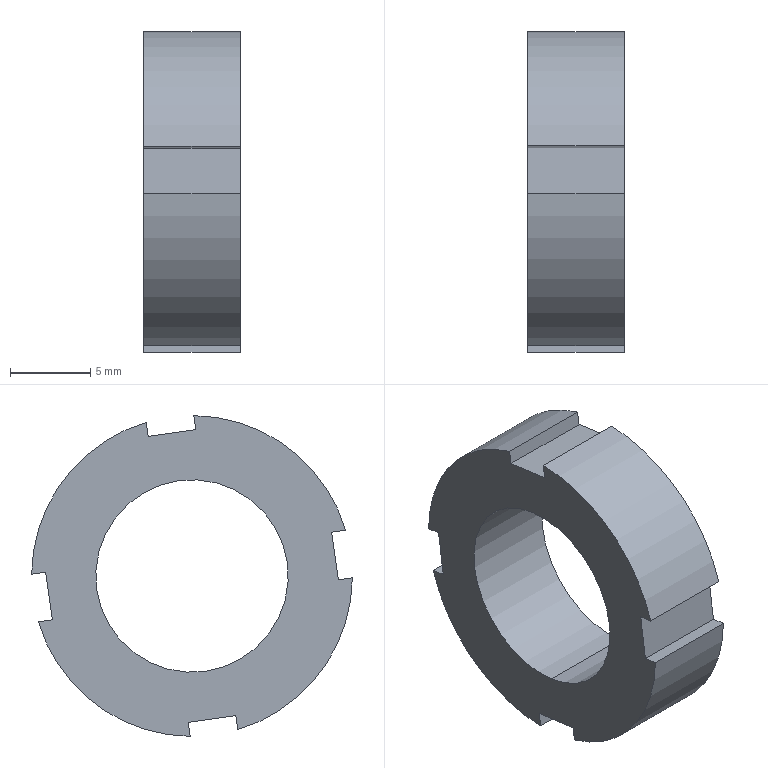Component | SolidWorks | ElectricalBoxAssembly2-1_RoundNut-1 | 1 solid | 20 faces | box 6 x 20 x 20 mm | volume 1137 mm3 | plane 14 | cylinder 6 | commonest cylinder face diameters 20 x4 12 x2
STEP:
#1=COLOUR_RGB('',0.7922,0.8196,0.9333);
#2=FILL_AREA_STYLE_COLOUR('',#1);
#3=FILL_AREA_STYLE('',(#2));
#4=SURFACE_STYLE_FILL_AREA(#3);
#5=SURFACE_SIDE_STYLE('',(#4));
#6=SURFACE_STYLE_USAGE(.BOTH.,#5);
#7=PRESENTATION_STYLE_ASSIGNMENT((#6));
#8=CARTESIAN_POINT('',(29.585,8.484,66.234));
#9=VERTEX_POINT('',#8);
#10=CARTESIAN_POINT('',(29.585,8.419,65.766));
#11=VERTEX_POINT('',#10);
#12=CARTESIAN_POINT('',(29.585,8.451,66.));
#13=DIRECTION('',(-1.,-0.,-0.));
#14=DIRECTION('',(0.,-0.1386,-0.9903));
#15=AXIS2_PLACEMENT_3D('',#12,#13,#14);
#16=CIRCLE('',#15,0.2362);
#17=EDGE_CURVE('',#9,#11,#16,.T.);
#18=ORIENTED_EDGE('',*,*,#17,.T.);
#19=CARTESIAN_POINT('',(29.822,8.419,65.766));
#20=VERTEX_POINT('',#19);
#21=CARTESIAN_POINT('',(29.585,8.419,65.766));
#22=DIRECTION('',(1.,0.,0.));
#23=VECTOR('',#22,39.37);
#24=LINE('',#21,#23);
#25=EDGE_CURVE('',#11,#20,#24,.T.);
#26=ORIENTED_EDGE('',*,*,#25,.T.);
#27=CARTESIAN_POINT('',(29.822,8.484,66.234));
#28=VERTEX_POINT('',#27);
#29=CARTESIAN_POINT('',(29.822,8.451,66.));
#30=DIRECTION('',(-1.,-0.,-0.));
#31=DIRECTION('',(0.,-0.1386,-0.9903));
#32=AXIS2_PLACEMENT_3D('',#29,#30,#31);
#33=CIRCLE('',#32,0.2362);
#34=EDGE_CURVE('',#28,#20,#33,.T.);
#35=ORIENTED_EDGE('',*,*,#34,.F.);
#36=CARTESIAN_POINT('',(29.585,8.484,66.234));
#37=DIRECTION('',(1.,0.,0.));
#38=VECTOR('',#37,39.37);
#39=LINE('',#36,#38);
#40=EDGE_CURVE('',#9,#28,#39,.T.);
#41=ORIENTED_EDGE('',*,*,#40,.F.);
#42=EDGE_LOOP('',(#18,#26,#35,#41));
#43=FACE_OUTER_BOUND('',#42,.T.);
#44=CARTESIAN_POINT('',(29.585,8.451,66.));
#45=DIRECTION('',(1.,0.,0.));
#46=DIRECTION('',(0.,0.1386,0.9903));
#47=AXIS2_PLACEMENT_3D('',#44,#45,#46);
#48=CYLINDRICAL_SURFACE('',#47,0.2362);
#49=ADVANCED_FACE('',(#43),#48,.F.);
#50=CARTESIAN_POINT('',(29.822,8.564,66.377));
#51=VERTEX_POINT('',#50);
#52=CARTESIAN_POINT('',(29.822,8.845,66.004));
#53=VERTEX_POINT('',#52);
#54=CARTESIAN_POINT('',(29.822,8.451,66.));
#55=DIRECTION('',(-1.,-0.,-0.));
#56=DIRECTION('',(0.,-0.1386,-0.9903));
#57=AXIS2_PLACEMENT_3D('',#54,#55,#56);
#58=CIRCLE('',#57,0.3937);
#59=EDGE_CURVE('',#51,#53,#58,.T.);
#60=ORIENTED_EDGE('',*,*,#59,.T.);
#61=CARTESIAN_POINT('',(29.585,8.845,66.004));
#62=VERTEX_POINT('',#61);
#63=CARTESIAN_POINT('',(29.585,8.845,66.004));
#64=DIRECTION('',(-1.,-0.,-0.));
#65=VECTOR('',#64,39.37);
#66=LINE('',#63,#65);
#67=EDGE_CURVE('',#53,#62,#66,.T.);
#68=ORIENTED_EDGE('',*,*,#67,.T.);
#69=CARTESIAN_POINT('',(29.585,8.564,66.377));
#70=VERTEX_POINT('',#69);
#71=CARTESIAN_POINT('',(29.585,8.451,66.));
#72=DIRECTION('',(-1.,-0.,-0.));
#73=DIRECTION('',(0.,-0.1386,-0.9903));
#74=AXIS2_PLACEMENT_3D('',#71,#72,#73);
#75=CIRCLE('',#74,0.3937);
#76=EDGE_CURVE('',#70,#62,#75,.T.);
#77=ORIENTED_EDGE('',*,*,#76,.F.);
#78=CARTESIAN_POINT('',(29.585,8.564,66.377));
#79=DIRECTION('',(1.,0.,0.));
#80=VECTOR('',#79,39.37);
#81=LINE('',#78,#80);
#82=EDGE_CURVE('',#70,#51,#81,.T.);
#83=ORIENTED_EDGE('',*,*,#82,.T.);
#84=EDGE_LOOP('',(#60,#68,#77,#83));
#85=FACE_OUTER_BOUND('',#84,.T.);
#86=CARTESIAN_POINT('',(29.585,8.451,66.));
#87=DIRECTION('',(1.,0.,0.));
#88=DIRECTION('',(0.,0.1386,0.9903));
#89=AXIS2_PLACEMENT_3D('',#86,#87,#88);
#90=CYLINDRICAL_SURFACE('',#89,0.3937);
#91=ADVANCED_FACE('',(#85),#90,.T.);
#92=CARTESIAN_POINT('',(29.822,8.074,66.112));
#93=VERTEX_POINT('',#92);
#94=CARTESIAN_POINT('',(29.822,8.447,66.394));
#95=VERTEX_POINT('',#94);
#96=CARTESIAN_POINT('',(29.822,8.451,66.));
#97=DIRECTION('',(-1.,-0.,-0.));
#98=DIRECTION('',(0.,-0.1386,-0.9903));
#99=AXIS2_PLACEMENT_3D('',#96,#97,#98);
#100=CIRCLE('',#99,0.3937);
#101=EDGE_CURVE('',#93,#95,#100,.T.);
#102=ORIENTED_EDGE('',*,*,#101,.T.);
#103=CARTESIAN_POINT('',(29.585,8.447,66.394));
#104=VERTEX_POINT('',#103);
#105=CARTESIAN_POINT('',(29.585,8.447,66.394));
#106=DIRECTION('',(-1.,-0.,-0.));
#107=VECTOR('',#106,39.37);
#108=LINE('',#105,#107);
#109=EDGE_CURVE('',#95,#104,#108,.T.);
#110=ORIENTED_EDGE('',*,*,#109,.T.);
#111=CARTESIAN_POINT('',(29.585,8.074,66.112));
#112=VERTEX_POINT('',#111);
#113=CARTESIAN_POINT('',(29.585,8.451,66.));
#114=DIRECTION('',(-1.,-0.,-0.));
#115=DIRECTION('',(0.,-0.1386,-0.9903));
#116=AXIS2_PLACEMENT_3D('',#113,#114,#115);
#117=CIRCLE('',#116,0.3937);
#118=EDGE_CURVE('',#112,#104,#117,.T.);
#119=ORIENTED_EDGE('',*,*,#118,.F.);
#120=CARTESIAN_POINT('',(29.585,8.074,66.112));
#121=DIRECTION('',(1.,0.,0.));
#122=VECTOR('',#121,39.37);
#123=LINE('',#120,#122);
#124=EDGE_CURVE('',#112,#93,#123,.T.);
#125=ORIENTED_EDGE('',*,*,#124,.T.);
#126=EDGE_LOOP('',(#102,#110,#119,#125));
#127=FACE_OUTER_BOUND('',#126,.T.);
#128=CARTESIAN_POINT('',(29.585,8.451,66.));
#129=DIRECTION('',(1.,0.,0.));
#130=DIRECTION('',(0.,0.1386,0.9903));
#131=AXIS2_PLACEMENT_3D('',#128,#129,#130);
#132=CYLINDRICAL_SURFACE('',#131,0.3937);
#133=ADVANCED_FACE('',(#127),#132,.T.);
#134=CARTESIAN_POINT('',(29.585,8.829,65.888));
#135=VERTEX_POINT('',#134);
#136=CARTESIAN_POINT('',(29.585,8.456,65.606));
#137=VERTEX_POINT('',#136);
#138=CARTESIAN_POINT('',(29.585,8.451,66.));
#139=DIRECTION('',(-1.,-0.,-0.));
#140=DIRECTION('',(0.,-0.1386,-0.9903));
#141=AXIS2_PLACEMENT_3D('',#138,#139,#140);
#142=CIRCLE('',#141,0.3937);
#143=EDGE_CURVE('',#135,#137,#142,.T.);
#144=ORIENTED_EDGE('',*,*,#143,.F.);
#145=CARTESIAN_POINT('',(29.822,8.829,65.888));
#146=VERTEX_POINT('',#145);
#147=CARTESIAN_POINT('',(29.585,8.829,65.888));
#148=DIRECTION('',(1.,0.,0.));
#149=VECTOR('',#148,39.37);
#150=LINE('',#147,#149);
#151=EDGE_CURVE('',#135,#146,#150,.T.);
#152=ORIENTED_EDGE('',*,*,#151,.T.);
#153=CARTESIAN_POINT('',(29.822,8.456,65.606));
#154=VERTEX_POINT('',#153);
#155=CARTESIAN_POINT('',(29.822,8.451,66.));
#156=DIRECTION('',(-1.,-0.,-0.));
#157=DIRECTION('',(0.,-0.1386,-0.9903));
#158=AXIS2_PLACEMENT_3D('',#155,#156,#157);
#159=CIRCLE('',#158,0.3937);
#160=EDGE_CURVE('',#146,#154,#159,.T.);
#161=ORIENTED_EDGE('',*,*,#160,.T.);
#162=CARTESIAN_POINT('',(29.585,8.456,65.606));
#163=DIRECTION('',(-1.,-0.,-0.));
#164=VECTOR('',#163,39.37);
#165=LINE('',#162,#164);
#166=EDGE_CURVE('',#154,#137,#165,.T.);
#167=ORIENTED_EDGE('',*,*,#166,.T.);
#168=EDGE_LOOP('',(#144,#152,#161,#167));
#169=FACE_OUTER_BOUND('',#168,.T.);
#170=CARTESIAN_POINT('',(29.585,8.451,66.));
#171=DIRECTION('',(1.,0.,0.));
#172=DIRECTION('',(0.,0.1386,0.9903));
#173=AXIS2_PLACEMENT_3D('',#170,#171,#172);
#174=CYLINDRICAL_SURFACE('',#173,0.3937);
#175=ADVANCED_FACE('',(#169),#174,.T.);
#176=CARTESIAN_POINT('',(29.585,8.811,66.009));
#177=VERTEX_POINT('',#176);
#178=CARTESIAN_POINT('',(29.585,8.888,65.998));
#179=DIRECTION('',(0.,0.9903,-0.1386));
#180=VECTOR('',#179,39.37);
#181=LINE('',#178,#180);
#182=EDGE_CURVE('',#177,#62,#181,.T.);
#183=ORIENTED_EDGE('',*,*,#182,.F.);
#184=CARTESIAN_POINT('',(29.585,8.794,65.892));
#185=VERTEX_POINT('',#184);
#186=CARTESIAN_POINT('',(29.585,8.794,65.892));
#187=DIRECTION('',(-0.,0.1386,0.9903));
#188=VECTOR('',#187,39.37);
#189=LINE('',#186,#188);
#190=EDGE_CURVE('',#185,#177,#189,.T.);
#191=ORIENTED_EDGE('',*,*,#190,.F.);
#192=CARTESIAN_POINT('',(29.585,8.872,65.881));
#193=DIRECTION('',(-0.,-0.9903,0.1386));
#194=VECTOR('',#193,39.37);
#195=LINE('',#192,#194);
#196=EDGE_CURVE('',#135,#185,#195,.T.);
#197=ORIENTED_EDGE('',*,*,#196,.F.);
#198=ORIENTED_EDGE('',*,*,#143,.T.);
#199=CARTESIAN_POINT('',(29.585,8.461,65.641));
#200=VERTEX_POINT('',#199);
#201=CARTESIAN_POINT('',(29.585,8.45,65.563));
#202=DIRECTION('',(0.,-0.1386,-0.9903));
#203=VECTOR('',#202,39.37);
#204=LINE('',#201,#203);
#205=EDGE_CURVE('',#200,#137,#204,.T.);
#206=ORIENTED_EDGE('',*,*,#205,.F.);
#207=CARTESIAN_POINT('',(29.585,8.344,65.657));
#208=VERTEX_POINT('',#207);
#209=CARTESIAN_POINT('',(29.585,8.344,65.657));
#210=DIRECTION('',(0.,0.9903,-0.1386));
#211=VECTOR('',#210,39.37);
#212=LINE('',#209,#211);
#213=EDGE_CURVE('',#208,#200,#212,.T.);
#214=ORIENTED_EDGE('',*,*,#213,.F.);
#215=CARTESIAN_POINT('',(29.585,8.339,65.623));
#216=VERTEX_POINT('',#215);
#217=CARTESIAN_POINT('',(29.585,8.333,65.579));
#218=DIRECTION('',(-0.,0.1386,0.9903));
#219=VECTOR('',#218,39.37);
#220=LINE('',#217,#219);
#221=EDGE_CURVE('',#216,#208,#220,.T.);
#222=ORIENTED_EDGE('',*,*,#221,.F.);
#223=CARTESIAN_POINT('',(29.585,8.058,65.995));
#224=VERTEX_POINT('',#223);
#225=CARTESIAN_POINT('',(29.585,8.451,66.));
#226=DIRECTION('',(-1.,-0.,-0.));
#227=DIRECTION('',(0.,-0.1386,-0.9903));
#228=AXIS2_PLACEMENT_3D('',#225,#226,#227);
#229=CIRCLE('',#228,0.3937);
#230=EDGE_CURVE('',#216,#224,#229,.T.);
#231=ORIENTED_EDGE('',*,*,#230,.T.);
#232=CARTESIAN_POINT('',(29.585,8.092,65.991));
#233=VERTEX_POINT('',#232);
#234=CARTESIAN_POINT('',(29.585,8.014,66.001));
#235=DIRECTION('',(-0.,-0.9903,0.1386));
#236=VECTOR('',#235,39.37);
#237=LINE('',#234,#236);
#238=EDGE_CURVE('',#233,#224,#237,.T.);
#239=ORIENTED_EDGE('',*,*,#238,.F.);
#240=CARTESIAN_POINT('',(29.585,8.109,66.108));
#241=VERTEX_POINT('',#240);
#242=CARTESIAN_POINT('',(29.585,8.109,66.108));
#243=DIRECTION('',(0.,-0.1386,-0.9903));
#244=VECTOR('',#243,39.37);
#245=LINE('',#242,#244);
#246=EDGE_CURVE('',#241,#233,#245,.T.);
#247=ORIENTED_EDGE('',*,*,#246,.F.);
#248=CARTESIAN_POINT('',(29.585,8.031,66.118));
#249=DIRECTION('',(0.,0.9903,-0.1386));
#250=VECTOR('',#249,39.37);
#251=LINE('',#248,#250);
#252=EDGE_CURVE('',#112,#241,#251,.T.);
#253=ORIENTED_EDGE('',*,*,#252,.F.);
#254=ORIENTED_EDGE('',*,*,#118,.T.);
#255=CARTESIAN_POINT('',(29.585,8.442,66.359));
#256=VERTEX_POINT('',#255);
#257=CARTESIAN_POINT('',(29.585,8.453,66.437));
#258=DIRECTION('',(-0.,0.1386,0.9903));
#259=VECTOR('',#258,39.37);
#260=LINE('',#257,#259);
#261=EDGE_CURVE('',#256,#104,#260,.T.);
#262=ORIENTED_EDGE('',*,*,#261,.F.);
#263=CARTESIAN_POINT('',(29.585,8.559,66.343));
#264=VERTEX_POINT('',#263);
#265=CARTESIAN_POINT('',(29.585,8.559,66.343));
#266=DIRECTION('',(-0.,-0.9903,0.1386));
#267=VECTOR('',#266,39.37);
#268=LINE('',#265,#267);
#269=EDGE_CURVE('',#264,#256,#268,.T.);
#270=ORIENTED_EDGE('',*,*,#269,.F.);
#271=CARTESIAN_POINT('',(29.585,8.57,66.421));
#272=DIRECTION('',(0.,-0.1386,-0.9903));
#273=VECTOR('',#272,39.37);
#274=LINE('',#271,#273);
#275=EDGE_CURVE('',#70,#264,#274,.T.);
#276=ORIENTED_EDGE('',*,*,#275,.F.);
#277=ORIENTED_EDGE('',*,*,#76,.T.);
#278=EDGE_LOOP('',(#183,#191,#197,#198,#206,#214,#222,#231,#239,#247,#253,#254,#262,#270,#276,#277));
#279=FACE_OUTER_BOUND('',#278,.T.);
#280=ORIENTED_EDGE('',*,*,#17,.F.);
#281=CARTESIAN_POINT('',(29.585,8.451,66.));
#282=DIRECTION('',(-1.,-0.,-0.));
#283=DIRECTION('',(0.,-0.1386,-0.9903));
#284=AXIS2_PLACEMENT_3D('',#281,#282,#283);
#285=CIRCLE('',#284,0.2362);
#286=EDGE_CURVE('',#11,#9,#285,.T.);
#287=ORIENTED_EDGE('',*,*,#286,.F.);
#288=EDGE_LOOP('',(#280,#287));
#289=FACE_BOUND('',#288,.T.);
#290=CARTESIAN_POINT('',(29.585,8.451,66.));
#291=DIRECTION('',(-1.,-0.,-0.));
#292=DIRECTION('',(0.,-0.1386,-0.9903));
#293=AXIS2_PLACEMENT_3D('',#290,#291,#292);
#294=PLANE('',#293);
#295=ADVANCED_FACE('',(#279,#289),#294,.T.);
#296=CARTESIAN_POINT('',(29.822,8.794,65.892));
#297=VERTEX_POINT('',#296);
#298=CARTESIAN_POINT('',(29.822,8.811,66.009));
#299=VERTEX_POINT('',#298);
#300=CARTESIAN_POINT('',(29.822,8.794,65.892));
#301=DIRECTION('',(-0.,0.1386,0.9903));
#302=VECTOR('',#301,39.37);
#303=LINE('',#300,#302);
#304=EDGE_CURVE('',#297,#299,#303,.T.);
#305=ORIENTED_EDGE('',*,*,#304,.T.);
#306=CARTESIAN_POINT('',(29.822,8.888,65.998));
#307=DIRECTION('',(0.,0.9903,-0.1386));
#308=VECTOR('',#307,39.37);
#309=LINE('',#306,#308);
#310=EDGE_CURVE('',#299,#53,#309,.T.);
#311=ORIENTED_EDGE('',*,*,#310,.T.);
#312=ORIENTED_EDGE('',*,*,#59,.F.);
#313=CARTESIAN_POINT('',(29.822,8.559,66.343));
#314=VERTEX_POINT('',#313);
#315=CARTESIAN_POINT('',(29.822,8.51,65.992));
#316=DIRECTION('',(0.,-0.1386,-0.9903));
#317=VECTOR('',#316,39.37);
#318=LINE('',#315,#317);
#319=EDGE_CURVE('',#51,#314,#318,.T.);
#320=ORIENTED_EDGE('',*,*,#319,.T.);
#321=CARTESIAN_POINT('',(29.822,8.442,66.359));
#322=VERTEX_POINT('',#321);
#323=CARTESIAN_POINT('',(29.822,8.559,66.343));
#324=DIRECTION('',(-0.,-0.9903,0.1386));
#325=VECTOR('',#324,39.37);
#326=LINE('',#323,#325);
#327=EDGE_CURVE('',#314,#322,#326,.T.);
#328=ORIENTED_EDGE('',*,*,#327,.T.);
#329=CARTESIAN_POINT('',(29.822,8.453,66.437));
#330=DIRECTION('',(-0.,0.1386,0.9903));
#331=VECTOR('',#330,39.37);
#332=LINE('',#329,#331);
#333=EDGE_CURVE('',#322,#95,#332,.T.);
#334=ORIENTED_EDGE('',*,*,#333,.T.);
#335=ORIENTED_EDGE('',*,*,#101,.F.);
#336=CARTESIAN_POINT('',(29.822,8.109,66.108));
#337=VERTEX_POINT('',#336);
#338=CARTESIAN_POINT('',(29.822,8.031,66.118));
#339=DIRECTION('',(0.,0.9903,-0.1386));
#340=VECTOR('',#339,39.37);
#341=LINE('',#338,#340);
#342=EDGE_CURVE('',#93,#337,#341,.T.);
#343=ORIENTED_EDGE('',*,*,#342,.T.);
#344=CARTESIAN_POINT('',(29.822,8.092,65.991));
#345=VERTEX_POINT('',#344);
#346=CARTESIAN_POINT('',(29.822,8.109,66.108));
#347=DIRECTION('',(0.,-0.1386,-0.9903));
#348=VECTOR('',#347,39.37);
#349=LINE('',#346,#348);
#350=EDGE_CURVE('',#337,#345,#349,.T.);
#351=ORIENTED_EDGE('',*,*,#350,.T.);
#352=CARTESIAN_POINT('',(29.822,8.058,65.995));
#353=VERTEX_POINT('',#352);
#354=CARTESIAN_POINT('',(29.822,8.014,66.001));
#355=DIRECTION('',(-0.,-0.9903,0.1386));
#356=VECTOR('',#355,39.37);
#357=LINE('',#354,#356);
#358=EDGE_CURVE('',#345,#353,#357,.T.);
#359=ORIENTED_EDGE('',*,*,#358,.T.);
#360=CARTESIAN_POINT('',(29.822,8.339,65.623));
#361=VERTEX_POINT('',#360);
#362=CARTESIAN_POINT('',(29.822,8.451,66.));
#363=DIRECTION('',(-1.,-0.,-0.));
#364=DIRECTION('',(0.,-0.1386,-0.9903));
#365=AXIS2_PLACEMENT_3D('',#362,#363,#364);
#366=CIRCLE('',#365,0.3937);
#367=EDGE_CURVE('',#361,#353,#366,.T.);
#368=ORIENTED_EDGE('',*,*,#367,.F.);
#369=CARTESIAN_POINT('',(29.822,8.344,65.657));
#370=VERTEX_POINT('',#369);
#371=CARTESIAN_POINT('',(29.822,8.333,65.579));
#372=DIRECTION('',(-0.,0.1386,0.9903));
#373=VECTOR('',#372,39.37);
#374=LINE('',#371,#373);
#375=EDGE_CURVE('',#361,#370,#374,.T.);
#376=ORIENTED_EDGE('',*,*,#375,.T.);
#377=CARTESIAN_POINT('',(29.822,8.461,65.641));
#378=VERTEX_POINT('',#377);
#379=CARTESIAN_POINT('',(29.822,8.344,65.657));
#380=DIRECTION('',(0.,0.9903,-0.1386));
#381=VECTOR('',#380,39.37);
#382=LINE('',#379,#381);
#383=EDGE_CURVE('',#370,#378,#382,.T.);
#384=ORIENTED_EDGE('',*,*,#383,.T.);
#385=CARTESIAN_POINT('',(29.822,8.45,65.563));
#386=DIRECTION('',(0.,-0.1386,-0.9903));
#387=VECTOR('',#386,39.37);
#388=LINE('',#385,#387);
#389=EDGE_CURVE('',#378,#154,#388,.T.);
#390=ORIENTED_EDGE('',*,*,#389,.T.);
#391=ORIENTED_EDGE('',*,*,#160,.F.);
#392=CARTESIAN_POINT('',(29.822,8.443,65.941));
#393=DIRECTION('',(-0.,-0.9903,0.1386));
#394=VECTOR('',#393,39.37);
#395=LINE('',#392,#394);
#396=EDGE_CURVE('',#146,#297,#395,.T.);
#397=ORIENTED_EDGE('',*,*,#396,.T.);
#398=EDGE_LOOP('',(#305,#311,#312,#320,#328,#334,#335,#343,#351,#359,#368,#376,#384,#390,#391,#397));
#399=FACE_OUTER_BOUND('',#398,.T.);
#400=ORIENTED_EDGE('',*,*,#34,.T.);
#401=CARTESIAN_POINT('',(29.822,8.451,66.));
#402=DIRECTION('',(-1.,-0.,-0.));
#403=DIRECTION('',(0.,-0.1386,-0.9903));
#404=AXIS2_PLACEMENT_3D('',#401,#402,#403);
#405=CIRCLE('',#404,0.2362);
#406=EDGE_CURVE('',#20,#28,#405,.T.);
#407=ORIENTED_EDGE('',*,*,#406,.T.);
#408=EDGE_LOOP('',(#400,#407));
#409=FACE_BOUND('',#408,.T.);
#410=CARTESIAN_POINT('',(29.822,8.451,66.));
#411=DIRECTION('',(-1.,-0.,-0.));
#412=DIRECTION('',(0.,-0.1386,-0.9903));
#413=AXIS2_PLACEMENT_3D('',#410,#411,#412);
#414=PLANE('',#413);
#415=ADVANCED_FACE('',(#399,#409),#414,.F.);
#416=ORIENTED_EDGE('',*,*,#230,.F.);
#417=CARTESIAN_POINT('',(29.585,8.339,65.623));
#418=DIRECTION('',(1.,0.,0.));
#419=VECTOR('',#418,39.37);
#420=LINE('',#417,#419);
#421=EDGE_CURVE('',#216,#361,#420,.T.);
#422=ORIENTED_EDGE('',*,*,#421,.T.);
#423=ORIENTED_EDGE('',*,*,#367,.T.);
#424=CARTESIAN_POINT('',(29.585,8.058,65.995));
#425=DIRECTION('',(-1.,-0.,-0.));
#426=VECTOR('',#425,39.37);
#427=LINE('',#424,#426);
#428=EDGE_CURVE('',#353,#224,#427,.T.);
#429=ORIENTED_EDGE('',*,*,#428,.T.);
#430=EDGE_LOOP('',(#416,#422,#423,#429));
#431=FACE_OUTER_BOUND('',#430,.T.);
#432=CARTESIAN_POINT('',(29.585,8.451,66.));
#433=DIRECTION('',(1.,0.,0.));
#434=DIRECTION('',(0.,0.1386,0.9903));
#435=AXIS2_PLACEMENT_3D('',#432,#433,#434);
#436=CYLINDRICAL_SURFACE('',#435,0.3937);
#437=ADVANCED_FACE('',(#431),#436,.T.);
#438=ORIENTED_EDGE('',*,*,#25,.F.);
#439=ORIENTED_EDGE('',*,*,#286,.T.);
#440=ORIENTED_EDGE('',*,*,#40,.T.);
#441=ORIENTED_EDGE('',*,*,#406,.F.);
#442=EDGE_LOOP('',(#438,#439,#440,#441));
#443=FACE_OUTER_BOUND('',#442,.T.);
#444=CARTESIAN_POINT('',(29.585,8.451,66.));
#445=DIRECTION('',(1.,0.,0.));
#446=DIRECTION('',(0.,0.1386,0.9903));
#447=AXIS2_PLACEMENT_3D('',#444,#445,#446);
#448=CYLINDRICAL_SURFACE('',#447,0.2362);
#449=ADVANCED_FACE('',(#443),#448,.F.);
#450=ORIENTED_EDGE('',*,*,#358,.F.);
#451=CARTESIAN_POINT('',(29.822,8.092,65.991));
#452=DIRECTION('',(-1.,-0.,-0.));
#453=VECTOR('',#452,39.37);
#454=LINE('',#451,#453);
#455=EDGE_CURVE('',#345,#233,#454,.T.);
#456=ORIENTED_EDGE('',*,*,#455,.T.);
#457=ORIENTED_EDGE('',*,*,#238,.T.);
#458=ORIENTED_EDGE('',*,*,#428,.F.);
#459=EDGE_LOOP('',(#450,#456,#457,#458));
#460=FACE_OUTER_BOUND('',#459,.T.);
#461=CARTESIAN_POINT('',(29.822,8.014,66.001));
#462=DIRECTION('',(0.,-0.1386,-0.9903));
#463=DIRECTION('',(-0.,-0.9903,0.1386));
#464=AXIS2_PLACEMENT_3D('',#461,#462,#463);
#465=PLANE('',#464);
#466=ADVANCED_FACE('',(#460),#465,.F.);
#467=ORIENTED_EDGE('',*,*,#252,.T.);
#468=CARTESIAN_POINT('',(29.822,8.109,66.108));
#469=DIRECTION('',(-1.,-0.,-0.));
#470=VECTOR('',#469,39.37);
#471=LINE('',#468,#470);
#472=EDGE_CURVE('',#337,#241,#471,.T.);
#473=ORIENTED_EDGE('',*,*,#472,.F.);
#474=ORIENTED_EDGE('',*,*,#342,.F.);
#475=ORIENTED_EDGE('',*,*,#124,.F.);
#476=EDGE_LOOP('',(#467,#473,#474,#475));
#477=FACE_OUTER_BOUND('',#476,.T.);
#478=CARTESIAN_POINT('',(29.822,8.031,66.118));
#479=DIRECTION('',(-0.,0.1386,0.9903));
#480=DIRECTION('',(-1.,-0.,-0.));
#481=AXIS2_PLACEMENT_3D('',#478,#479,#480);
#482=PLANE('',#481);
#483=ADVANCED_FACE('',(#477),#482,.F.);
#484=ORIENTED_EDGE('',*,*,#455,.F.);
#485=ORIENTED_EDGE('',*,*,#350,.F.);
#486=ORIENTED_EDGE('',*,*,#472,.T.);
#487=ORIENTED_EDGE('',*,*,#246,.T.);
#488=EDGE_LOOP('',(#484,#485,#486,#487));
#489=FACE_OUTER_BOUND('',#488,.T.);
#490=CARTESIAN_POINT('',(29.822,8.109,66.108));
#491=DIRECTION('',(0.,0.9903,-0.1386));
#492=DIRECTION('',(1.,0.,0.));
#493=AXIS2_PLACEMENT_3D('',#490,#491,#492);
#494=PLANE('',#493);
#495=ADVANCED_FACE('',(#489),#494,.F.);
#496=ORIENTED_EDGE('',*,*,#389,.F.);
#497=CARTESIAN_POINT('',(29.822,8.461,65.641));
#498=DIRECTION('',(-1.,-0.,-0.));
#499=VECTOR('',#498,39.37);
#500=LINE('',#497,#499);
#501=EDGE_CURVE('',#378,#200,#500,.T.);
#502=ORIENTED_EDGE('',*,*,#501,.T.);
#503=ORIENTED_EDGE('',*,*,#205,.T.);
#504=ORIENTED_EDGE('',*,*,#166,.F.);
#505=EDGE_LOOP('',(#496,#502,#503,#504));
#506=FACE_OUTER_BOUND('',#505,.T.);
#507=CARTESIAN_POINT('',(29.822,8.45,65.563));
#508=DIRECTION('',(0.,0.9903,-0.1386));
#509=DIRECTION('',(0.,-0.1386,-0.9903));
#510=AXIS2_PLACEMENT_3D('',#507,#508,#509);
#511=PLANE('',#510);
#512=ADVANCED_FACE('',(#506),#511,.F.);
#513=ORIENTED_EDGE('',*,*,#221,.T.);
#514=CARTESIAN_POINT('',(29.822,8.344,65.657));
#515=DIRECTION('',(-1.,-0.,-0.));
#516=VECTOR('',#515,39.37);
#517=LINE('',#514,#516);
#518=EDGE_CURVE('',#370,#208,#517,.T.);
#519=ORIENTED_EDGE('',*,*,#518,.F.);
#520=ORIENTED_EDGE('',*,*,#375,.F.);
#521=ORIENTED_EDGE('',*,*,#421,.F.);
#522=EDGE_LOOP('',(#513,#519,#520,#521));
#523=FACE_OUTER_BOUND('',#522,.T.);
#524=CARTESIAN_POINT('',(29.822,8.333,65.579));
#525=DIRECTION('',(-0.,-0.9903,0.1386));
#526=DIRECTION('',(-0.,0.1386,0.9903));
#527=AXIS2_PLACEMENT_3D('',#524,#525,#526);
#528=PLANE('',#527);
#529=ADVANCED_FACE('',(#523),#528,.F.);
#530=ORIENTED_EDGE('',*,*,#501,.F.);
#531=ORIENTED_EDGE('',*,*,#383,.F.);
#532=ORIENTED_EDGE('',*,*,#518,.T.);
#533=ORIENTED_EDGE('',*,*,#213,.T.);
#534=EDGE_LOOP('',(#530,#531,#532,#533));
#535=FACE_OUTER_BOUND('',#534,.T.);
#536=CARTESIAN_POINT('',(29.822,8.344,65.657));
#537=DIRECTION('',(-0.,0.1386,0.9903));
#538=DIRECTION('',(0.,0.9903,-0.1386));
#539=AXIS2_PLACEMENT_3D('',#536,#537,#538);
#540=PLANE('',#539);
#541=ADVANCED_FACE('',(#535),#540,.F.);
#542=ORIENTED_EDGE('',*,*,#333,.F.);
#543=CARTESIAN_POINT('',(29.822,8.442,66.359));
#544=DIRECTION('',(-1.,-0.,-0.));
#545=VECTOR('',#544,39.37);
#546=LINE('',#543,#545);
#547=EDGE_CURVE('',#322,#256,#546,.T.);
#548=ORIENTED_EDGE('',*,*,#547,.T.);
#549=ORIENTED_EDGE('',*,*,#261,.T.);
#550=ORIENTED_EDGE('',*,*,#109,.F.);
#551=EDGE_LOOP('',(#542,#548,#549,#550));
#552=FACE_OUTER_BOUND('',#551,.T.);
#553=CARTESIAN_POINT('',(29.822,8.453,66.437));
#554=DIRECTION('',(-0.,-0.9903,0.1386));
#555=DIRECTION('',(-0.,0.1386,0.9903));
#556=AXIS2_PLACEMENT_3D('',#553,#554,#555);
#557=PLANE('',#556);
#558=ADVANCED_FACE('',(#552),#557,.F.);
#559=ORIENTED_EDGE('',*,*,#275,.T.);
#560=CARTESIAN_POINT('',(29.822,8.559,66.343));
#561=DIRECTION('',(-1.,-0.,-0.));
#562=VECTOR('',#561,39.37);
#563=LINE('',#560,#562);
#564=EDGE_CURVE('',#314,#264,#563,.T.);
#565=ORIENTED_EDGE('',*,*,#564,.F.);
#566=ORIENTED_EDGE('',*,*,#319,.F.);
#567=ORIENTED_EDGE('',*,*,#82,.F.);
#568=EDGE_LOOP('',(#559,#565,#566,#567));
#569=FACE_OUTER_BOUND('',#568,.T.);
#570=CARTESIAN_POINT('',(29.822,8.57,66.421));
#571=DIRECTION('',(0.,0.9903,-0.1386));
#572=DIRECTION('',(0.,-0.1386,-0.9903));
#573=AXIS2_PLACEMENT_3D('',#570,#571,#572);
#574=PLANE('',#573);
#575=ADVANCED_FACE('',(#569),#574,.F.);
#576=ORIENTED_EDGE('',*,*,#547,.F.);
#577=ORIENTED_EDGE('',*,*,#327,.F.);
#578=ORIENTED_EDGE('',*,*,#564,.T.);
#579=ORIENTED_EDGE('',*,*,#269,.T.);
#580=EDGE_LOOP('',(#576,#577,#578,#579));
#581=FACE_OUTER_BOUND('',#580,.T.);
#582=CARTESIAN_POINT('',(29.822,8.559,66.343));
#583=DIRECTION('',(0.,-0.1386,-0.9903));
#584=DIRECTION('',(-0.,-0.9903,0.1386));
#585=AXIS2_PLACEMENT_3D('',#582,#583,#584);
#586=PLANE('',#585);
#587=ADVANCED_FACE('',(#581),#586,.F.);
#588=ORIENTED_EDGE('',*,*,#310,.F.);
#589=CARTESIAN_POINT('',(29.822,8.811,66.009));
#590=DIRECTION('',(-1.,-0.,-0.));
#591=VECTOR('',#590,39.37);
#592=LINE('',#589,#591);
#593=EDGE_CURVE('',#299,#177,#592,.T.);
#594=ORIENTED_EDGE('',*,*,#593,.T.);
#595=ORIENTED_EDGE('',*,*,#182,.T.);
#596=ORIENTED_EDGE('',*,*,#67,.F.);
#597=EDGE_LOOP('',(#588,#594,#595,#596));
#598=FACE_OUTER_BOUND('',#597,.T.);
#599=CARTESIAN_POINT('',(29.822,8.888,65.998));
#600=DIRECTION('',(-0.,0.1386,0.9903));
#601=DIRECTION('',(0.,0.9903,-0.1386));
#602=AXIS2_PLACEMENT_3D('',#599,#600,#601);
#603=PLANE('',#602);
#604=ADVANCED_FACE('',(#598),#603,.F.);
#605=ORIENTED_EDGE('',*,*,#196,.T.);
#606=CARTESIAN_POINT('',(29.822,8.794,65.892));
#607=DIRECTION('',(-1.,-0.,-0.));
#608=VECTOR('',#607,39.37);
#609=LINE('',#606,#608);
#610=EDGE_CURVE('',#297,#185,#609,.T.);
#611=ORIENTED_EDGE('',*,*,#610,.F.);
#612=ORIENTED_EDGE('',*,*,#396,.F.);
#613=ORIENTED_EDGE('',*,*,#151,.F.);
#614=EDGE_LOOP('',(#605,#611,#612,#613));
#615=FACE_OUTER_BOUND('',#614,.T.);
#616=CARTESIAN_POINT('',(29.822,8.872,65.881));
#617=DIRECTION('',(0.,-0.1386,-0.9903));
#618=DIRECTION('',(1.,0.,0.));
#619=AXIS2_PLACEMENT_3D('',#616,#617,#618);
#620=PLANE('',#619);
#621=ADVANCED_FACE('',(#615),#620,.F.);
#622=ORIENTED_EDGE('',*,*,#593,.F.);
#623=ORIENTED_EDGE('',*,*,#304,.F.);
#624=ORIENTED_EDGE('',*,*,#610,.T.);
#625=ORIENTED_EDGE('',*,*,#190,.T.);
#626=EDGE_LOOP('',(#622,#623,#624,#625));
#627=FACE_OUTER_BOUND('',#626,.T.);
#628=CARTESIAN_POINT('',(29.822,8.794,65.892));
#629=DIRECTION('',(-0.,-0.9903,0.1386));
#630=DIRECTION('',(-1.,-0.,-0.));
#631=AXIS2_PLACEMENT_3D('',#628,#629,#630);
#632=PLANE('',#631);
#633=ADVANCED_FACE('',(#627),#632,.F.);
#634=CLOSED_SHELL('',(#49,#91,#133,#175,#295,#415,#437,#449,#466,#483,#495,#512,#529,#541,#558,#575,#587,#604,#621,#633));
#635=MANIFOLD_SOLID_BREP('',#634);
#636=STYLED_ITEM('',(#7),#635);
#637=PRESENTATION_LAYER_ASSIGNMENT('','',(#636));
#638=(LENGTH_UNIT()NAMED_UNIT(*)SI_UNIT($,.METRE.));
#639=LENGTH_MEASURE_WITH_UNIT(LENGTH_MEASURE(0.0254),#638);
#640=DIMENSIONAL_EXPONENTS(1.,0.,0.,0.,0.,0.,0.);
#641=(CONVERSION_BASED_UNIT('',#639)LENGTH_UNIT()NAMED_UNIT(#640));
#642=UNCERTAINTY_MEASURE_WITH_UNIT(LENGTH_MEASURE(0.00001),#641,'','');
#643=(NAMED_UNIT(*)PLANE_ANGLE_UNIT()SI_UNIT($,.RADIAN.));
#644=(NAMED_UNIT(*)SI_UNIT($,.STERADIAN.)SOLID_ANGLE_UNIT());
#645=(GEOMETRIC_REPRESENTATION_CONTEXT(3)GLOBAL_UNCERTAINTY_ASSIGNED_CONTEXT((#642))GLOBAL_UNIT_ASSIGNED_CONTEXT((#641,#643,#644))REPRESENTATION_CONTEXT('',''));
#646=MECHANICAL_DESIGN_GEOMETRIC_PRESENTATION_REPRESENTATION('',(#636),#645);
#647=CARTESIAN_POINT('',(0.,0.,0.));
#648=DIRECTION('',(0.,0.,1.));
#649=DIRECTION('',(1.,0.,0.));
#650=AXIS2_PLACEMENT_3D('',#647,#648,#649);
#651=(LENGTH_UNIT()NAMED_UNIT(*)SI_UNIT($,.METRE.));
#652=LENGTH_MEASURE_WITH_UNIT(LENGTH_MEASURE(0.0254),#651);
#653=DIMENSIONAL_EXPONENTS(1.,0.,0.,0.,0.,0.,0.);
#654=(CONVERSION_BASED_UNIT('',#652)LENGTH_UNIT()NAMED_UNIT(#653));
#655=UNCERTAINTY_MEASURE_WITH_UNIT(LENGTH_MEASURE(0.00001),#654,'','');
#656=(NAMED_UNIT(*)PLANE_ANGLE_UNIT()SI_UNIT($,.RADIAN.));
#657=(NAMED_UNIT(*)SI_UNIT($,.STERADIAN.)SOLID_ANGLE_UNIT());
#658=(GEOMETRIC_REPRESENTATION_CONTEXT(3)GLOBAL_UNCERTAINTY_ASSIGNED_CONTEXT((#655))GLOBAL_UNIT_ASSIGNED_CONTEXT((#654,#656,#657))REPRESENTATION_CONTEXT('',''));
#659=ADVANCED_BREP_SHAPE_REPRESENTATION('',(#635,#650),#658);